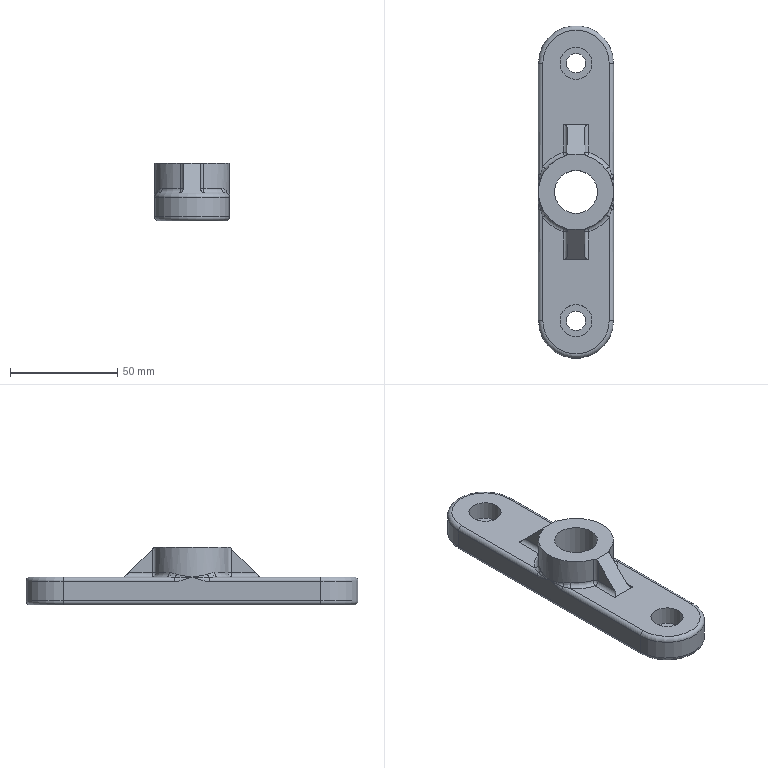Component | NX | FIXED_PLATE | 1 solid | 61 faces | volume 69596 mm3 | cylinder 23 | plane 14 | spline 12 | torus 8 | sphere 4 | commonest cylinder face diameters 4 x14 35 x4 9 x2 15 x2 20 x1